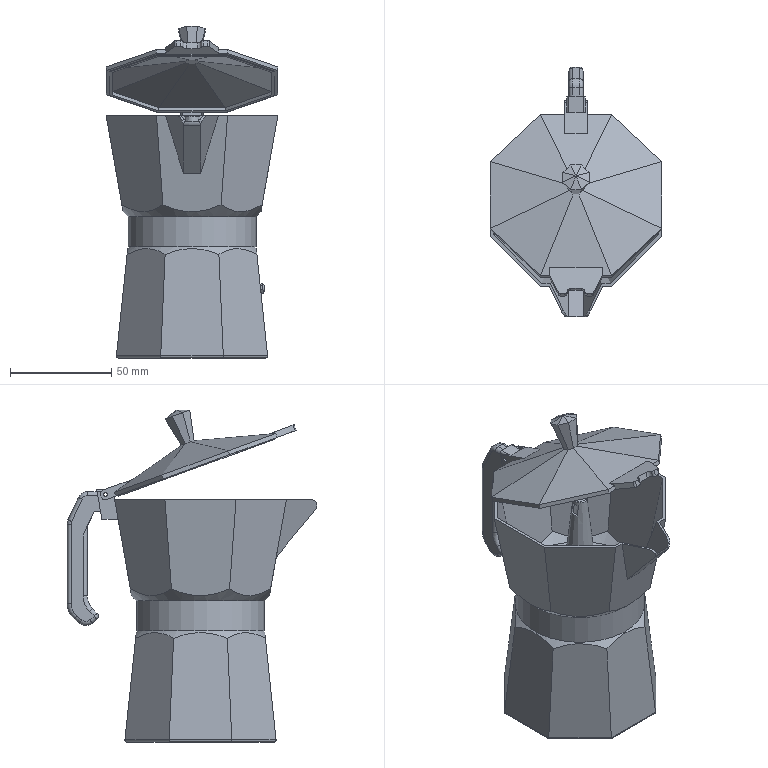Assembly | NX | mm | 6 component files | 6 solids | 462 faces | box 85 x 123.68 x 164.29 mm | volume 74763 mm3 | cylinder 255 | plane 171 | torus 21 | cone 11 | sphere 2 | other 2 | commonest cylinder face diameters 1 x200 4 x21 2 x16 10 x3 60 x2 62 x2 20 x1 17.901 x1
Bill of materials:
unnamed part 1 | 1 |  | Funnel-shaped revolved part: a short open cylindrical cup with a thin lip at the rim and a flat perforated floor, a conical transition below it, and a narrow cylindrical tube at the bottom with a rounded end.
unnamed part 2 | 1 |  | Elongated solid bar with a rectangular, rounded-edge cross-section, bent into a shallow C/hook profile: a long straight middle section, an angled flat-faced head at one end, and a curved rounded tail at the other end.
unnamed part 3 | 1 |  | Thin octagonal lid-like shell with a low faceted pyramidal top that rises to a small central flat. A rim runs around the underside, a notched tab sticks out from one edge, and a pair of thin parallel lugs with a small hole sticks out from the opposite edge.
unnamed part 4 | 1 |  | Solid octagonal tapered prism (truncated pyramid-like frustum) with a low eight-facet pyramidal cap on the wider end and a flat octagonal face on the narrower end.
unnamed part 5 | 1 |  | Open vessel with faceted octagonal walls that flare outward toward the top. It has a pointed pouring spout on one side, a small flat tab with a hole on the opposite side, and a cylindrical neck at the bottom. Inside, a central tapered tube rises from a conical boss on the floor.
unnamed part 6 | 1 |  | Octagonal tapered container body with a wide flat base and a cylindrical collar at the narrower top. A thin rim sits at the collar opening, and a small faceted boss with a central hole sticks out from one side face.
Mates:
1. touch align | model27 1 face | model26 1 face
2. concentric | model25 1 edge | model26 1 edge
3. touch align | model28 1 face | model25 1 face
4. touch align | model25 1 face | model23 1 edge
5. concentric | model25 1 edge | model23 1 edge
6. concentric | model24 1 edge | model23 1 edge
7. fix | model23 1 component
8. touch align | model26 1 edge | model27 1 edge